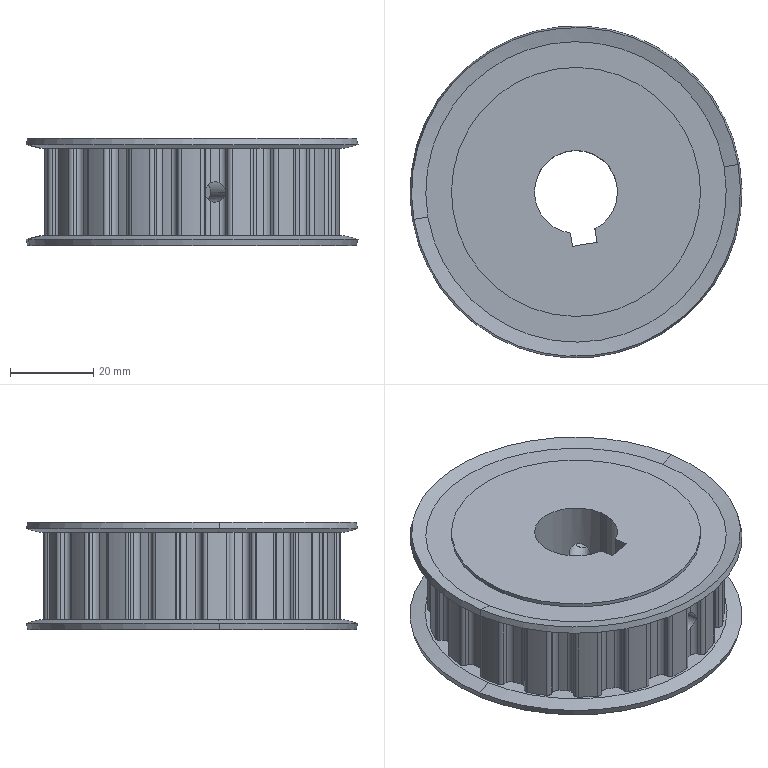Component | SolidWorks | ATPA18H075-A-N20-1_-2-1 | 1 solid | 195 faces | volume 90710 mm3 | cylinder 137 | plane 46 | cone 12 | commonest cylinder face diameters 2.94 x43 2.08 x42 66.21 x20 71.39 x19 60 x4 4.917 x4 20 x3 5.02 x2